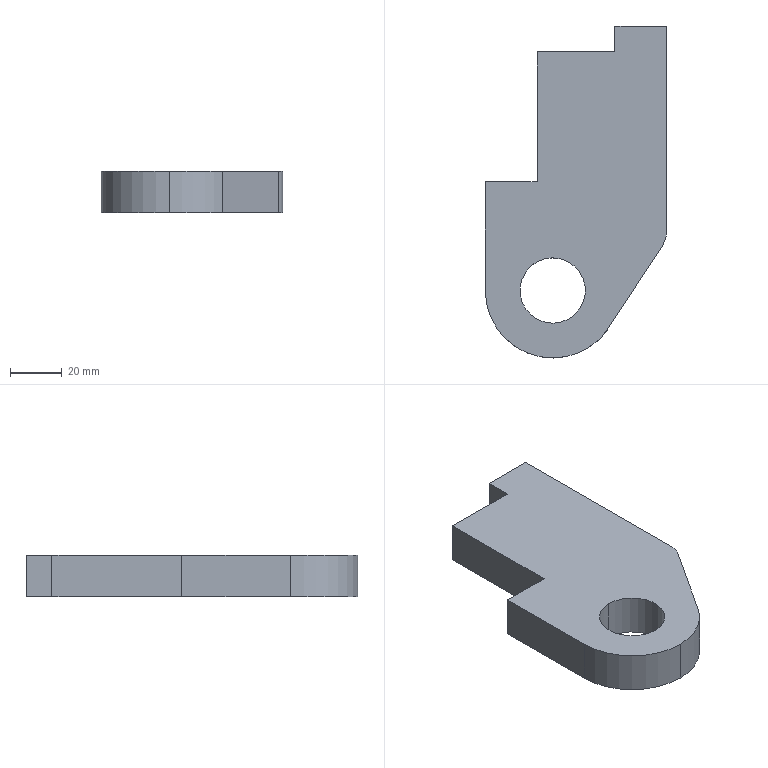Component | SolidWorks | VehicleBodyLowerLug-1 | 1 solid | 15 faces | box 70 x 128 x 16 mm | volume 97551 mm3 | plane 10 | cylinder 5 | commonest cylinder face diameters 25.2 x2 52 x2 20 x1 | material Q235
build123d program:
from build123d import *

# Parameters (mm, degrees)
SKETCH1_R           = 12.6
BOSS_EXTRUDE1_DEPTH = 16


with BuildPart() as part:
    # Sketch1 → Boss-Extrude1 (new body)
    with BuildSketch(Plane.XY):
        with BuildLine():
            Line((73.611, 4.283), (81.61, 4.361))
            Line((81.61, 4.361), (81.414, 24.36))
            Line((81.414, 24.36), (131.411, 24.851))
            Line((131.411, 24.851), (131.117, 54.85))
            Line((131.117, 54.85), (141.117, 54.948))
            Line((141.117, 54.948), (140.92, 74.947))
            Line((140.92, 74.947), (130.92, 74.849))
            Line((130.92, 74.849), (64.803, 74.2))
            Line((64.803, 74.2), (61.803, 74.17))
            ThreePointArc((61.803, 74.17), (59.028, 73.749), (56.479, 72.573))
            Line((56.479, 72.573), (23.562, 50.598))
            ThreePointArc((23.562, 50.598), (14.774, 21.488), (39.615, 3.949))
            Line((39.615, 3.949), (41.615, 3.969))
            Line((41.615, 3.969), (73.611, 4.283))
        make_face()
        with Locations((39.359, 29.948)):
            Circle(SKETCH1_R, mode=Mode.SUBTRACT)
    extrude(amount=BOSS_EXTRUDE1_DEPTH)


solid = part.part

# Placed as in the assembly
solid = solid.moved(Location((-1381.214, 1144.825, 2455.705), (180, 0, -90.563)))
STEP:
#1=CARTESIAN_POINT('',(-53.21,46.137,96.051));
#2=VERTEX_POINT('',#1);
#3=CARTESIAN_POINT('',(-53.22,47.129,96.051));
#4=VERTEX_POINT('',#3);
#5=CARTESIAN_POINT('',(-53.215,46.633,96.051));
#6=DIRECTION('',(-0.,-0.,-1.));
#7=DIRECTION('',(-0.009819,1.,0.));
#8=AXIS2_PLACEMENT_3D('',#5,#6,#7);
#9=CIRCLE('',#8,0.4961);
#10=EDGE_CURVE('',#2,#4,#9,.T.);
#11=ORIENTED_EDGE('',*,*,#10,.T.);
#12=CARTESIAN_POINT('',(-53.22,47.129,96.681));
#13=VERTEX_POINT('',#12);
#14=CARTESIAN_POINT('',(-53.22,47.129,96.051));
#15=DIRECTION('',(0.,0.,1.));
#16=VECTOR('',#15,39.37);
#17=LINE('',#14,#16);
#18=EDGE_CURVE('',#4,#13,#17,.T.);
#19=ORIENTED_EDGE('',*,*,#18,.T.);
#20=CARTESIAN_POINT('',(-53.21,46.137,96.681));
#21=VERTEX_POINT('',#20);
#22=CARTESIAN_POINT('',(-53.215,46.633,96.681));
#23=DIRECTION('',(-0.,-0.,-1.));
#24=DIRECTION('',(-0.009819,1.,0.));
#25=AXIS2_PLACEMENT_3D('',#22,#23,#24);
#26=CIRCLE('',#25,0.4961);
#27=EDGE_CURVE('',#21,#13,#26,.T.);
#28=ORIENTED_EDGE('',*,*,#27,.F.);
#29=CARTESIAN_POINT('',(-53.21,46.137,96.051));
#30=DIRECTION('',(0.,0.,1.));
#31=VECTOR('',#30,39.37);
#32=LINE('',#29,#31);
#33=EDGE_CURVE('',#2,#21,#32,.T.);
#34=ORIENTED_EDGE('',*,*,#33,.F.);
#35=EDGE_LOOP('',(#11,#19,#28,#34));
#36=FACE_OUTER_BOUND('',#35,.T.);
#37=CARTESIAN_POINT('',(-53.215,46.633,96.051));
#38=DIRECTION('',(0.,0.,1.));
#39=DIRECTION('',(0.009819,-1.,0.));
#40=AXIS2_PLACEMENT_3D('',#37,#38,#39);
#41=CYLINDRICAL_SURFACE('',#40,0.4961);
#42=ADVANCED_FACE('',(#36),#41,.F.);
#43=CARTESIAN_POINT('',(-53.205,45.609,96.051));
#44=VERTEX_POINT('',#43);
#45=CARTESIAN_POINT('',(-54.238,46.633,96.051));
#46=VERTEX_POINT('',#45);
#47=CARTESIAN_POINT('',(-53.215,46.633,96.051));
#48=DIRECTION('',(-0.,-0.,-1.));
#49=DIRECTION('',(-0.009819,1.,0.));
#50=AXIS2_PLACEMENT_3D('',#47,#48,#49);
#51=CIRCLE('',#50,1.024);
#52=EDGE_CURVE('',#44,#46,#51,.T.);
#53=ORIENTED_EDGE('',*,*,#52,.F.);
#54=CARTESIAN_POINT('',(-53.205,45.609,96.681));
#55=VERTEX_POINT('',#54);
#56=CARTESIAN_POINT('',(-53.205,45.609,96.051));
#57=DIRECTION('',(0.,0.,1.));
#58=VECTOR('',#57,39.37);
#59=LINE('',#56,#58);
#60=EDGE_CURVE('',#44,#55,#59,.T.);
#61=ORIENTED_EDGE('',*,*,#60,.T.);
#62=CARTESIAN_POINT('',(-54.238,46.633,96.681));
#63=VERTEX_POINT('',#62);
#64=CARTESIAN_POINT('',(-53.215,46.633,96.681));
#65=DIRECTION('',(-0.,-0.,-1.));
#66=DIRECTION('',(-0.009819,1.,0.));
#67=AXIS2_PLACEMENT_3D('',#64,#65,#66);
#68=CIRCLE('',#67,1.024);
#69=EDGE_CURVE('',#55,#63,#68,.T.);
#70=ORIENTED_EDGE('',*,*,#69,.T.);
#71=CARTESIAN_POINT('',(-54.238,46.633,96.051));
#72=DIRECTION('',(0.,0.,1.));
#73=VECTOR('',#72,39.37);
#74=LINE('',#71,#73);
#75=EDGE_CURVE('',#46,#63,#74,.T.);
#76=ORIENTED_EDGE('',*,*,#75,.F.);
#77=EDGE_LOOP('',(#53,#61,#70,#76));
#78=FACE_OUTER_BOUND('',#77,.T.);
#79=CARTESIAN_POINT('',(-53.215,46.633,96.051));
#80=DIRECTION('',(0.,0.,1.));
#81=DIRECTION('',(0.009819,-1.,0.));
#82=AXIS2_PLACEMENT_3D('',#79,#80,#81);
#83=CYLINDRICAL_SURFACE('',#82,1.024);
#84=ADVANCED_FACE('',(#78),#83,.T.);
#85=CARTESIAN_POINT('',(-51.482,47.534,96.681));
#86=VERTEX_POINT('',#85);
#87=CARTESIAN_POINT('',(-51.482,50.649,96.681));
#88=VERTEX_POINT('',#87);
#89=CARTESIAN_POINT('',(-51.482,45.072,96.681));
#90=DIRECTION('',(-0.,1.,-0.));
#91=VECTOR('',#90,39.37);
#92=LINE('',#89,#91);
#93=EDGE_CURVE('',#86,#88,#92,.T.);
#94=ORIENTED_EDGE('',*,*,#93,.F.);
#95=CARTESIAN_POINT('',(-51.482,47.534,96.051));
#96=VERTEX_POINT('',#95);
#97=CARTESIAN_POINT('',(-51.482,47.534,96.051));
#98=DIRECTION('',(0.,0.,1.));
#99=VECTOR('',#98,39.37);
#100=LINE('',#97,#99);
#101=EDGE_CURVE('',#96,#86,#100,.T.);
#102=ORIENTED_EDGE('',*,*,#101,.F.);
#103=CARTESIAN_POINT('',(-51.482,50.649,96.051));
#104=VERTEX_POINT('',#103);
#105=CARTESIAN_POINT('',(-51.482,45.072,96.051));
#106=DIRECTION('',(-0.,1.,-0.));
#107=VECTOR('',#106,39.37);
#108=LINE('',#105,#107);
#109=EDGE_CURVE('',#96,#104,#108,.T.);
#110=ORIENTED_EDGE('',*,*,#109,.T.);
#111=CARTESIAN_POINT('',(-51.482,50.649,96.051));
#112=DIRECTION('',(0.,0.,1.));
#113=VECTOR('',#112,39.37);
#114=LINE('',#111,#113);
#115=EDGE_CURVE('',#104,#88,#114,.T.);
#116=ORIENTED_EDGE('',*,*,#115,.T.);
#117=EDGE_LOOP('',(#94,#102,#110,#116));
#118=FACE_OUTER_BOUND('',#117,.T.);
#119=CARTESIAN_POINT('',(-51.482,45.072,96.051));
#120=DIRECTION('',(1.,0.,-0.));
#121=DIRECTION('',(0.,-1.,0.));
#122=AXIS2_PLACEMENT_3D('',#119,#120,#121);
#123=PLANE('',#122);
#124=ADVANCED_FACE('',(#118),#123,.T.);
#125=CARTESIAN_POINT('',(-51.543,47.323,96.681));
#126=VERTEX_POINT('',#125);
#127=CARTESIAN_POINT('',(-51.876,47.534,96.681));
#128=DIRECTION('',(-0.,-0.,-1.));
#129=DIRECTION('',(-0.009819,1.,0.));
#130=AXIS2_PLACEMENT_3D('',#127,#128,#129);
#131=CIRCLE('',#130,0.3937);
#132=EDGE_CURVE('',#86,#126,#131,.T.);
#133=ORIENTED_EDGE('',*,*,#132,.T.);
#134=CARTESIAN_POINT('',(-51.543,47.323,96.051));
#135=VERTEX_POINT('',#134);
#136=CARTESIAN_POINT('',(-51.543,47.323,96.051));
#137=DIRECTION('',(0.,0.,1.));
#138=VECTOR('',#137,39.37);
#139=LINE('',#136,#138);
#140=EDGE_CURVE('',#135,#126,#139,.T.);
#141=ORIENTED_EDGE('',*,*,#140,.F.);
#142=CARTESIAN_POINT('',(-51.876,47.534,96.051));
#143=DIRECTION('',(-0.,-0.,-1.));
#144=DIRECTION('',(-0.009819,1.,0.));
#145=AXIS2_PLACEMENT_3D('',#142,#143,#144);
#146=CIRCLE('',#145,0.3937);
#147=EDGE_CURVE('',#96,#135,#146,.T.);
#148=ORIENTED_EDGE('',*,*,#147,.F.);
#149=ORIENTED_EDGE('',*,*,#101,.T.);
#150=EDGE_LOOP('',(#133,#141,#148,#149));
#151=FACE_OUTER_BOUND('',#150,.T.);
#152=CARTESIAN_POINT('',(-51.876,47.534,96.051));
#153=DIRECTION('',(0.,0.,1.));
#154=DIRECTION('',(0.009819,-1.,0.));
#155=AXIS2_PLACEMENT_3D('',#152,#153,#154);
#156=CYLINDRICAL_SURFACE('',#155,0.3937);
#157=ADVANCED_FACE('',(#151),#156,.T.);
#158=CARTESIAN_POINT('',(-52.396,46.019,96.681));
#159=VERTEX_POINT('',#158);
#160=CARTESIAN_POINT('',(-53.423,44.447,96.681));
#161=DIRECTION('',(0.547,0.8371,-0.));
#162=VECTOR('',#161,39.37);
#163=LINE('',#160,#162);
#164=EDGE_CURVE('',#159,#126,#163,.T.);
#165=ORIENTED_EDGE('',*,*,#164,.F.);
#166=CARTESIAN_POINT('',(-52.396,46.019,96.051));
#167=VERTEX_POINT('',#166);
#168=CARTESIAN_POINT('',(-52.396,46.019,96.051));
#169=DIRECTION('',(0.,0.,1.));
#170=VECTOR('',#169,39.37);
#171=LINE('',#168,#170);
#172=EDGE_CURVE('',#167,#159,#171,.T.);
#173=ORIENTED_EDGE('',*,*,#172,.F.);
#174=CARTESIAN_POINT('',(-53.423,44.447,96.051));
#175=DIRECTION('',(0.547,0.8371,-0.));
#176=VECTOR('',#175,39.37);
#177=LINE('',#174,#176);
#178=EDGE_CURVE('',#167,#135,#177,.T.);
#179=ORIENTED_EDGE('',*,*,#178,.T.);
#180=ORIENTED_EDGE('',*,*,#140,.T.);
#181=EDGE_LOOP('',(#165,#173,#179,#180));
#182=FACE_OUTER_BOUND('',#181,.T.);
#183=CARTESIAN_POINT('',(-53.423,44.447,96.051));
#184=DIRECTION('',(0.8371,-0.547,-0.));
#185=DIRECTION('',(-0.547,-0.8371,0.));
#186=AXIS2_PLACEMENT_3D('',#183,#184,#185);
#187=PLANE('',#186);
#188=ADVANCED_FACE('',(#182),#187,.T.);
#189=ORIENTED_EDGE('',*,*,#60,.F.);
#190=CARTESIAN_POINT('',(-53.215,46.633,96.051));
#191=DIRECTION('',(-0.,-0.,-1.));
#192=DIRECTION('',(-0.009819,1.,0.));
#193=AXIS2_PLACEMENT_3D('',#190,#191,#192);
#194=CIRCLE('',#193,1.024);
#195=EDGE_CURVE('',#167,#44,#194,.T.);
#196=ORIENTED_EDGE('',*,*,#195,.F.);
#197=ORIENTED_EDGE('',*,*,#172,.T.);
#198=CARTESIAN_POINT('',(-53.215,46.633,96.681));
#199=DIRECTION('',(-0.,-0.,-1.));
#200=DIRECTION('',(-0.009819,1.,0.));
#201=AXIS2_PLACEMENT_3D('',#198,#199,#200);
#202=CIRCLE('',#201,1.024);
#203=EDGE_CURVE('',#159,#55,#202,.T.);
#204=ORIENTED_EDGE('',*,*,#203,.T.);
#205=EDGE_LOOP('',(#189,#196,#197,#204));
#206=FACE_OUTER_BOUND('',#205,.T.);
#207=CARTESIAN_POINT('',(-53.215,46.633,96.051));
#208=DIRECTION('',(0.,0.,1.));
#209=DIRECTION('',(0.009819,-1.,0.));
#210=AXIS2_PLACEMENT_3D('',#207,#208,#209);
#211=CYLINDRICAL_SURFACE('',#210,1.024);
#212=ADVANCED_FACE('',(#206),#211,.T.);
#213=CARTESIAN_POINT('',(-54.238,48.286,96.681));
#214=VERTEX_POINT('',#213);
#215=CARTESIAN_POINT('',(-54.238,45.072,96.681));
#216=DIRECTION('',(0.,1.,-0.));
#217=VECTOR('',#216,39.37);
#218=LINE('',#215,#217);
#219=EDGE_CURVE('',#63,#214,#218,.T.);
#220=ORIENTED_EDGE('',*,*,#219,.T.);
#221=CARTESIAN_POINT('',(-54.238,48.286,96.051));
#222=VERTEX_POINT('',#221);
#223=CARTESIAN_POINT('',(-54.238,48.286,96.051));
#224=DIRECTION('',(0.,0.,1.));
#225=VECTOR('',#224,39.37);
#226=LINE('',#223,#225);
#227=EDGE_CURVE('',#222,#214,#226,.T.);
#228=ORIENTED_EDGE('',*,*,#227,.F.);
#229=CARTESIAN_POINT('',(-54.238,45.072,96.051));
#230=DIRECTION('',(0.,1.,-0.));
#231=VECTOR('',#230,39.37);
#232=LINE('',#229,#231);
#233=EDGE_CURVE('',#46,#222,#232,.T.);
#234=ORIENTED_EDGE('',*,*,#233,.F.);
#235=ORIENTED_EDGE('',*,*,#75,.T.);
#236=EDGE_LOOP('',(#220,#228,#234,#235));
#237=FACE_OUTER_BOUND('',#236,.T.);
#238=CARTESIAN_POINT('',(-54.238,45.072,96.051));
#239=DIRECTION('',(1.,-0.,-0.));
#240=DIRECTION('',(-0.,-1.,0.));
#241=AXIS2_PLACEMENT_3D('',#238,#239,#240);
#242=PLANE('',#241);
#243=ADVANCED_FACE('',(#237),#242,.F.);
#244=CARTESIAN_POINT('',(-53.451,48.286,96.681));
#245=VERTEX_POINT('',#244);
#246=CARTESIAN_POINT('',(-54.379,48.286,96.681));
#247=DIRECTION('',(1.,-0.,-0.));
#248=VECTOR('',#247,39.37);
#249=LINE('',#246,#248);
#250=EDGE_CURVE('',#214,#245,#249,.T.);
#251=ORIENTED_EDGE('',*,*,#250,.T.);
#252=CARTESIAN_POINT('',(-53.451,48.286,96.051));
#253=VERTEX_POINT('',#252);
#254=CARTESIAN_POINT('',(-53.451,48.286,96.051));
#255=DIRECTION('',(0.,0.,1.));
#256=VECTOR('',#255,39.37);
#257=LINE('',#254,#256);
#258=EDGE_CURVE('',#253,#245,#257,.T.);
#259=ORIENTED_EDGE('',*,*,#258,.F.);
#260=CARTESIAN_POINT('',(-54.379,48.286,96.051));
#261=DIRECTION('',(1.,-0.,-0.));
#262=VECTOR('',#261,39.37);
#263=LINE('',#260,#262);
#264=EDGE_CURVE('',#222,#253,#263,.T.);
#265=ORIENTED_EDGE('',*,*,#264,.F.);
#266=ORIENTED_EDGE('',*,*,#227,.T.);
#267=EDGE_LOOP('',(#251,#259,#265,#266));
#268=FACE_OUTER_BOUND('',#267,.T.);
#269=CARTESIAN_POINT('',(-54.379,48.286,96.051));
#270=DIRECTION('',(-0.,-1.,0.));
#271=DIRECTION('',(-1.,0.,0.));
#272=AXIS2_PLACEMENT_3D('',#269,#270,#271);
#273=PLANE('',#272);
#274=ADVANCED_FACE('',(#268),#273,.F.);
#275=CARTESIAN_POINT('',(-53.451,50.255,96.681));
#276=VERTEX_POINT('',#275);
#277=CARTESIAN_POINT('',(-53.451,45.072,96.681));
#278=DIRECTION('',(0.,1.,-0.));
#279=VECTOR('',#278,39.37);
#280=LINE('',#277,#279);
#281=EDGE_CURVE('',#245,#276,#280,.T.);
#282=ORIENTED_EDGE('',*,*,#281,.T.);
#283=CARTESIAN_POINT('',(-53.451,50.255,96.051));
#284=VERTEX_POINT('',#283);
#285=CARTESIAN_POINT('',(-53.451,50.255,96.051));
#286=DIRECTION('',(0.,0.,1.));
#287=VECTOR('',#286,39.37);
#288=LINE('',#285,#287);
#289=EDGE_CURVE('',#284,#276,#288,.T.);
#290=ORIENTED_EDGE('',*,*,#289,.F.);
#291=CARTESIAN_POINT('',(-53.451,45.072,96.051));
#292=DIRECTION('',(0.,1.,-0.));
#293=VECTOR('',#292,39.37);
#294=LINE('',#291,#293);
#295=EDGE_CURVE('',#253,#284,#294,.T.);
#296=ORIENTED_EDGE('',*,*,#295,.F.);
#297=ORIENTED_EDGE('',*,*,#258,.T.);
#298=EDGE_LOOP('',(#282,#290,#296,#297));
#299=FACE_OUTER_BOUND('',#298,.T.);
#300=CARTESIAN_POINT('',(-53.451,45.072,96.051));
#301=DIRECTION('',(1.,-0.,-0.));
#302=DIRECTION('',(-0.,-1.,0.));
#303=AXIS2_PLACEMENT_3D('',#300,#301,#302);
#304=PLANE('',#303);
#305=ADVANCED_FACE('',(#299),#304,.F.);
#306=CARTESIAN_POINT('',(-52.27,50.255,96.681));
#307=VERTEX_POINT('',#306);
#308=CARTESIAN_POINT('',(-54.379,50.255,96.681));
#309=DIRECTION('',(-1.,0.,0.));
#310=VECTOR('',#309,39.37);
#311=LINE('',#308,#310);
#312=EDGE_CURVE('',#307,#276,#311,.T.);
#313=ORIENTED_EDGE('',*,*,#312,.F.);
#314=CARTESIAN_POINT('',(-52.27,50.255,96.051));
#315=VERTEX_POINT('',#314);
#316=CARTESIAN_POINT('',(-52.27,50.255,96.051));
#317=DIRECTION('',(0.,0.,1.));
#318=VECTOR('',#317,39.37);
#319=LINE('',#316,#318);
#320=EDGE_CURVE('',#315,#307,#319,.T.);
#321=ORIENTED_EDGE('',*,*,#320,.F.);
#322=CARTESIAN_POINT('',(-54.379,50.255,96.051));
#323=DIRECTION('',(-1.,0.,0.));
#324=VECTOR('',#323,39.37);
#325=LINE('',#322,#324);
#326=EDGE_CURVE('',#315,#284,#325,.T.);
#327=ORIENTED_EDGE('',*,*,#326,.T.);
#328=ORIENTED_EDGE('',*,*,#289,.T.);
#329=EDGE_LOOP('',(#313,#321,#327,#328));
#330=FACE_OUTER_BOUND('',#329,.T.);
#331=CARTESIAN_POINT('',(-54.379,50.255,96.051));
#332=DIRECTION('',(0.,1.,-0.));
#333=DIRECTION('',(1.,-0.,-0.));
#334=AXIS2_PLACEMENT_3D('',#331,#332,#333);
#335=PLANE('',#334);
#336=ADVANCED_FACE('',(#330),#335,.T.);
#337=CARTESIAN_POINT('',(-52.27,50.649,96.681));
#338=VERTEX_POINT('',#337);
#339=CARTESIAN_POINT('',(-52.27,45.072,96.681));
#340=DIRECTION('',(-0.,-1.,0.));
#341=VECTOR('',#340,39.37);
#342=LINE('',#339,#341);
#343=EDGE_CURVE('',#338,#307,#342,.T.);
#344=ORIENTED_EDGE('',*,*,#343,.F.);
#345=CARTESIAN_POINT('',(-52.27,50.649,96.051));
#346=VERTEX_POINT('',#345);
#347=CARTESIAN_POINT('',(-52.27,50.649,96.051));
#348=DIRECTION('',(0.,0.,1.));
#349=VECTOR('',#348,39.37);
#350=LINE('',#347,#349);
#351=EDGE_CURVE('',#346,#338,#350,.T.);
#352=ORIENTED_EDGE('',*,*,#351,.F.);
#353=CARTESIAN_POINT('',(-52.27,45.072,96.051));
#354=DIRECTION('',(-0.,-1.,0.));
#355=VECTOR('',#354,39.37);
#356=LINE('',#353,#355);
#357=EDGE_CURVE('',#346,#315,#356,.T.);
#358=ORIENTED_EDGE('',*,*,#357,.T.);
#359=ORIENTED_EDGE('',*,*,#320,.T.);
#360=EDGE_LOOP('',(#344,#352,#358,#359));
#361=FACE_OUTER_BOUND('',#360,.T.);
#362=CARTESIAN_POINT('',(-52.27,45.072,96.051));
#363=DIRECTION('',(-1.,0.,0.));
#364=DIRECTION('',(0.,1.,-0.));
#365=AXIS2_PLACEMENT_3D('',#362,#363,#364);
#366=PLANE('',#365);
#367=ADVANCED_FACE('',(#361),#366,.T.);
#368=ORIENTED_EDGE('',*,*,#18,.F.);
#369=CARTESIAN_POINT('',(-53.215,46.633,96.051));
#370=DIRECTION('',(-0.,-0.,-1.));
#371=DIRECTION('',(-0.009819,1.,0.));
#372=AXIS2_PLACEMENT_3D('',#369,#370,#371);
#373=CIRCLE('',#372,0.4961);
#374=EDGE_CURVE('',#4,#2,#373,.T.);
#375=ORIENTED_EDGE('',*,*,#374,.T.);
#376=ORIENTED_EDGE('',*,*,#33,.T.);
#377=CARTESIAN_POINT('',(-53.215,46.633,96.681));
#378=DIRECTION('',(-0.,-0.,-1.));
#379=DIRECTION('',(-0.009819,1.,0.));
#380=AXIS2_PLACEMENT_3D('',#377,#378,#379);
#381=CIRCLE('',#380,0.4961);
#382=EDGE_CURVE('',#13,#21,#381,.T.);
#383=ORIENTED_EDGE('',*,*,#382,.F.);
#384=EDGE_LOOP('',(#368,#375,#376,#383));
#385=FACE_OUTER_BOUND('',#384,.T.);
#386=CARTESIAN_POINT('',(-53.215,46.633,96.051));
#387=DIRECTION('',(0.,0.,1.));
#388=DIRECTION('',(0.009819,-1.,0.));
#389=AXIS2_PLACEMENT_3D('',#386,#387,#388);
#390=CYLINDRICAL_SURFACE('',#389,0.4961);
#391=ADVANCED_FACE('',(#385),#390,.F.);
#392=CARTESIAN_POINT('',(-54.379,50.649,96.681));
#393=DIRECTION('',(-1.,0.,0.));
#394=VECTOR('',#393,39.37);
#395=LINE('',#392,#394);
#396=EDGE_CURVE('',#88,#338,#395,.T.);
#397=ORIENTED_EDGE('',*,*,#396,.F.);
#398=ORIENTED_EDGE('',*,*,#115,.F.);
#399=CARTESIAN_POINT('',(-54.379,50.649,96.051));
#400=DIRECTION('',(-1.,0.,0.));
#401=VECTOR('',#400,39.37);
#402=LINE('',#399,#401);
#403=EDGE_CURVE('',#104,#346,#402,.T.);
#404=ORIENTED_EDGE('',*,*,#403,.T.);
#405=ORIENTED_EDGE('',*,*,#351,.T.);
#406=EDGE_LOOP('',(#397,#398,#404,#405));
#407=FACE_OUTER_BOUND('',#406,.T.);
#408=CARTESIAN_POINT('',(-54.379,50.649,96.051));
#409=DIRECTION('',(0.,1.,-0.));
#410=DIRECTION('',(1.,-0.,-0.));
#411=AXIS2_PLACEMENT_3D('',#408,#409,#410);
#412=PLANE('',#411);
#413=ADVANCED_FACE('',(#407),#412,.T.);
#414=ORIENTED_EDGE('',*,*,#10,.F.);
#415=ORIENTED_EDGE('',*,*,#374,.F.);
#416=EDGE_LOOP('',(#414,#415));
#417=FACE_BOUND('',#416,.T.);
#418=ORIENTED_EDGE('',*,*,#109,.F.);
#419=ORIENTED_EDGE('',*,*,#147,.T.);
#420=ORIENTED_EDGE('',*,*,#178,.F.);
#421=ORIENTED_EDGE('',*,*,#195,.T.);
#422=ORIENTED_EDGE('',*,*,#52,.T.);
#423=ORIENTED_EDGE('',*,*,#233,.T.);
#424=ORIENTED_EDGE('',*,*,#264,.T.);
#425=ORIENTED_EDGE('',*,*,#295,.T.);
#426=ORIENTED_EDGE('',*,*,#326,.F.);
#427=ORIENTED_EDGE('',*,*,#357,.F.);
#428=ORIENTED_EDGE('',*,*,#403,.F.);
#429=EDGE_LOOP('',(#418,#419,#420,#421,#422,#423,#424,#425,#426,#427,#428));
#430=FACE_OUTER_BOUND('',#429,.T.);
#431=CARTESIAN_POINT('',(-54.379,45.072,96.051));
#432=DIRECTION('',(-0.,-0.,-1.));
#433=DIRECTION('',(-0.009819,1.,-0.));
#434=AXIS2_PLACEMENT_3D('',#431,#432,#433);
#435=PLANE('',#434);
#436=ADVANCED_FACE('',(#417,#430),#435,.T.);
#437=ORIENTED_EDGE('',*,*,#27,.T.);
#438=ORIENTED_EDGE('',*,*,#382,.T.);
#439=EDGE_LOOP('',(#437,#438));
#440=FACE_BOUND('',#439,.T.);
#441=ORIENTED_EDGE('',*,*,#93,.T.);
#442=ORIENTED_EDGE('',*,*,#396,.T.);
#443=ORIENTED_EDGE('',*,*,#343,.T.);
#444=ORIENTED_EDGE('',*,*,#312,.T.);
#445=ORIENTED_EDGE('',*,*,#281,.F.);
#446=ORIENTED_EDGE('',*,*,#250,.F.);
#447=ORIENTED_EDGE('',*,*,#219,.F.);
#448=ORIENTED_EDGE('',*,*,#69,.F.);
#449=ORIENTED_EDGE('',*,*,#203,.F.);
#450=ORIENTED_EDGE('',*,*,#164,.T.);
#451=ORIENTED_EDGE('',*,*,#132,.F.);
#452=EDGE_LOOP('',(#441,#442,#443,#444,#445,#446,#447,#448,#449,#450,#451));
#453=FACE_OUTER_BOUND('',#452,.T.);
#454=CARTESIAN_POINT('',(-54.379,45.072,96.681));
#455=DIRECTION('',(-0.,-0.,-1.));
#456=DIRECTION('',(-0.009819,1.,-0.));
#457=AXIS2_PLACEMENT_3D('',#454,#455,#456);
#458=PLANE('',#457);
#459=ADVANCED_FACE('',(#440,#453),#458,.F.);
#460=CLOSED_SHELL('',(#42,#84,#124,#157,#188,#212,#243,#274,#305,#336,#367,#391,#413,#436,#459));
#461=MANIFOLD_SOLID_BREP('',#460);
#462=CARTESIAN_POINT('',(0.,0.,0.));
#463=DIRECTION('',(0.,0.,1.));
#464=DIRECTION('',(1.,0.,0.));
#465=AXIS2_PLACEMENT_3D('',#462,#463,#464);
#466=(LENGTH_UNIT()NAMED_UNIT(*)SI_UNIT($,.METRE.));
#467=LENGTH_MEASURE_WITH_UNIT(LENGTH_MEASURE(0.0254),#466);
#468=DIMENSIONAL_EXPONENTS(1.,0.,0.,0.,0.,0.,0.);
#469=(CONVERSION_BASED_UNIT('',#467)LENGTH_UNIT()NAMED_UNIT(#468));
#470=UNCERTAINTY_MEASURE_WITH_UNIT(LENGTH_MEASURE(0.00001),#469,'','');
#471=(NAMED_UNIT(*)PLANE_ANGLE_UNIT()SI_UNIT($,.RADIAN.));
#472=(NAMED_UNIT(*)SI_UNIT($,.STERADIAN.)SOLID_ANGLE_UNIT());
#473=(GEOMETRIC_REPRESENTATION_CONTEXT(3)GLOBAL_UNCERTAINTY_ASSIGNED_CONTEXT((#470))GLOBAL_UNIT_ASSIGNED_CONTEXT((#469,#471,#472))REPRESENTATION_CONTEXT('',''));
#474=ADVANCED_BREP_SHAPE_REPRESENTATION('',(#461,#465),#473);
#475=COLOUR_RGB('',0.7922,0.8196,0.9333);
#476=FILL_AREA_STYLE_COLOUR('',#475);
#477=FILL_AREA_STYLE('',(#476));
#478=SURFACE_STYLE_FILL_AREA(#477);
#479=SURFACE_SIDE_STYLE('',(#478));
#480=SURFACE_STYLE_USAGE(.BOTH.,#479);
#481=PRESENTATION_STYLE_ASSIGNMENT((#480));
#482=STYLED_ITEM('',(#481),#461);
#483=PRESENTATION_LAYER_ASSIGNMENT('','',(#482));
#484=(LENGTH_UNIT()NAMED_UNIT(*)SI_UNIT($,.METRE.));
#485=LENGTH_MEASURE_WITH_UNIT(LENGTH_MEASURE(0.0254),#484);
#486=DIMENSIONAL_EXPONENTS(1.,0.,0.,0.,0.,0.,0.);
#487=(CONVERSION_BASED_UNIT('',#485)LENGTH_UNIT()NAMED_UNIT(#486));
#488=UNCERTAINTY_MEASURE_WITH_UNIT(LENGTH_MEASURE(0.00001),#487,'','');
#489=(NAMED_UNIT(*)PLANE_ANGLE_UNIT()SI_UNIT($,.RADIAN.));
#490=(NAMED_UNIT(*)SI_UNIT($,.STERADIAN.)SOLID_ANGLE_UNIT());
#491=(GEOMETRIC_REPRESENTATION_CONTEXT(3)GLOBAL_UNCERTAINTY_ASSIGNED_CONTEXT((#488))GLOBAL_UNIT_ASSIGNED_CONTEXT((#487,#489,#490))REPRESENTATION_CONTEXT('',''));
#492=MECHANICAL_DESIGN_GEOMETRIC_PRESENTATION_REPRESENTATION('',(#482),#491);